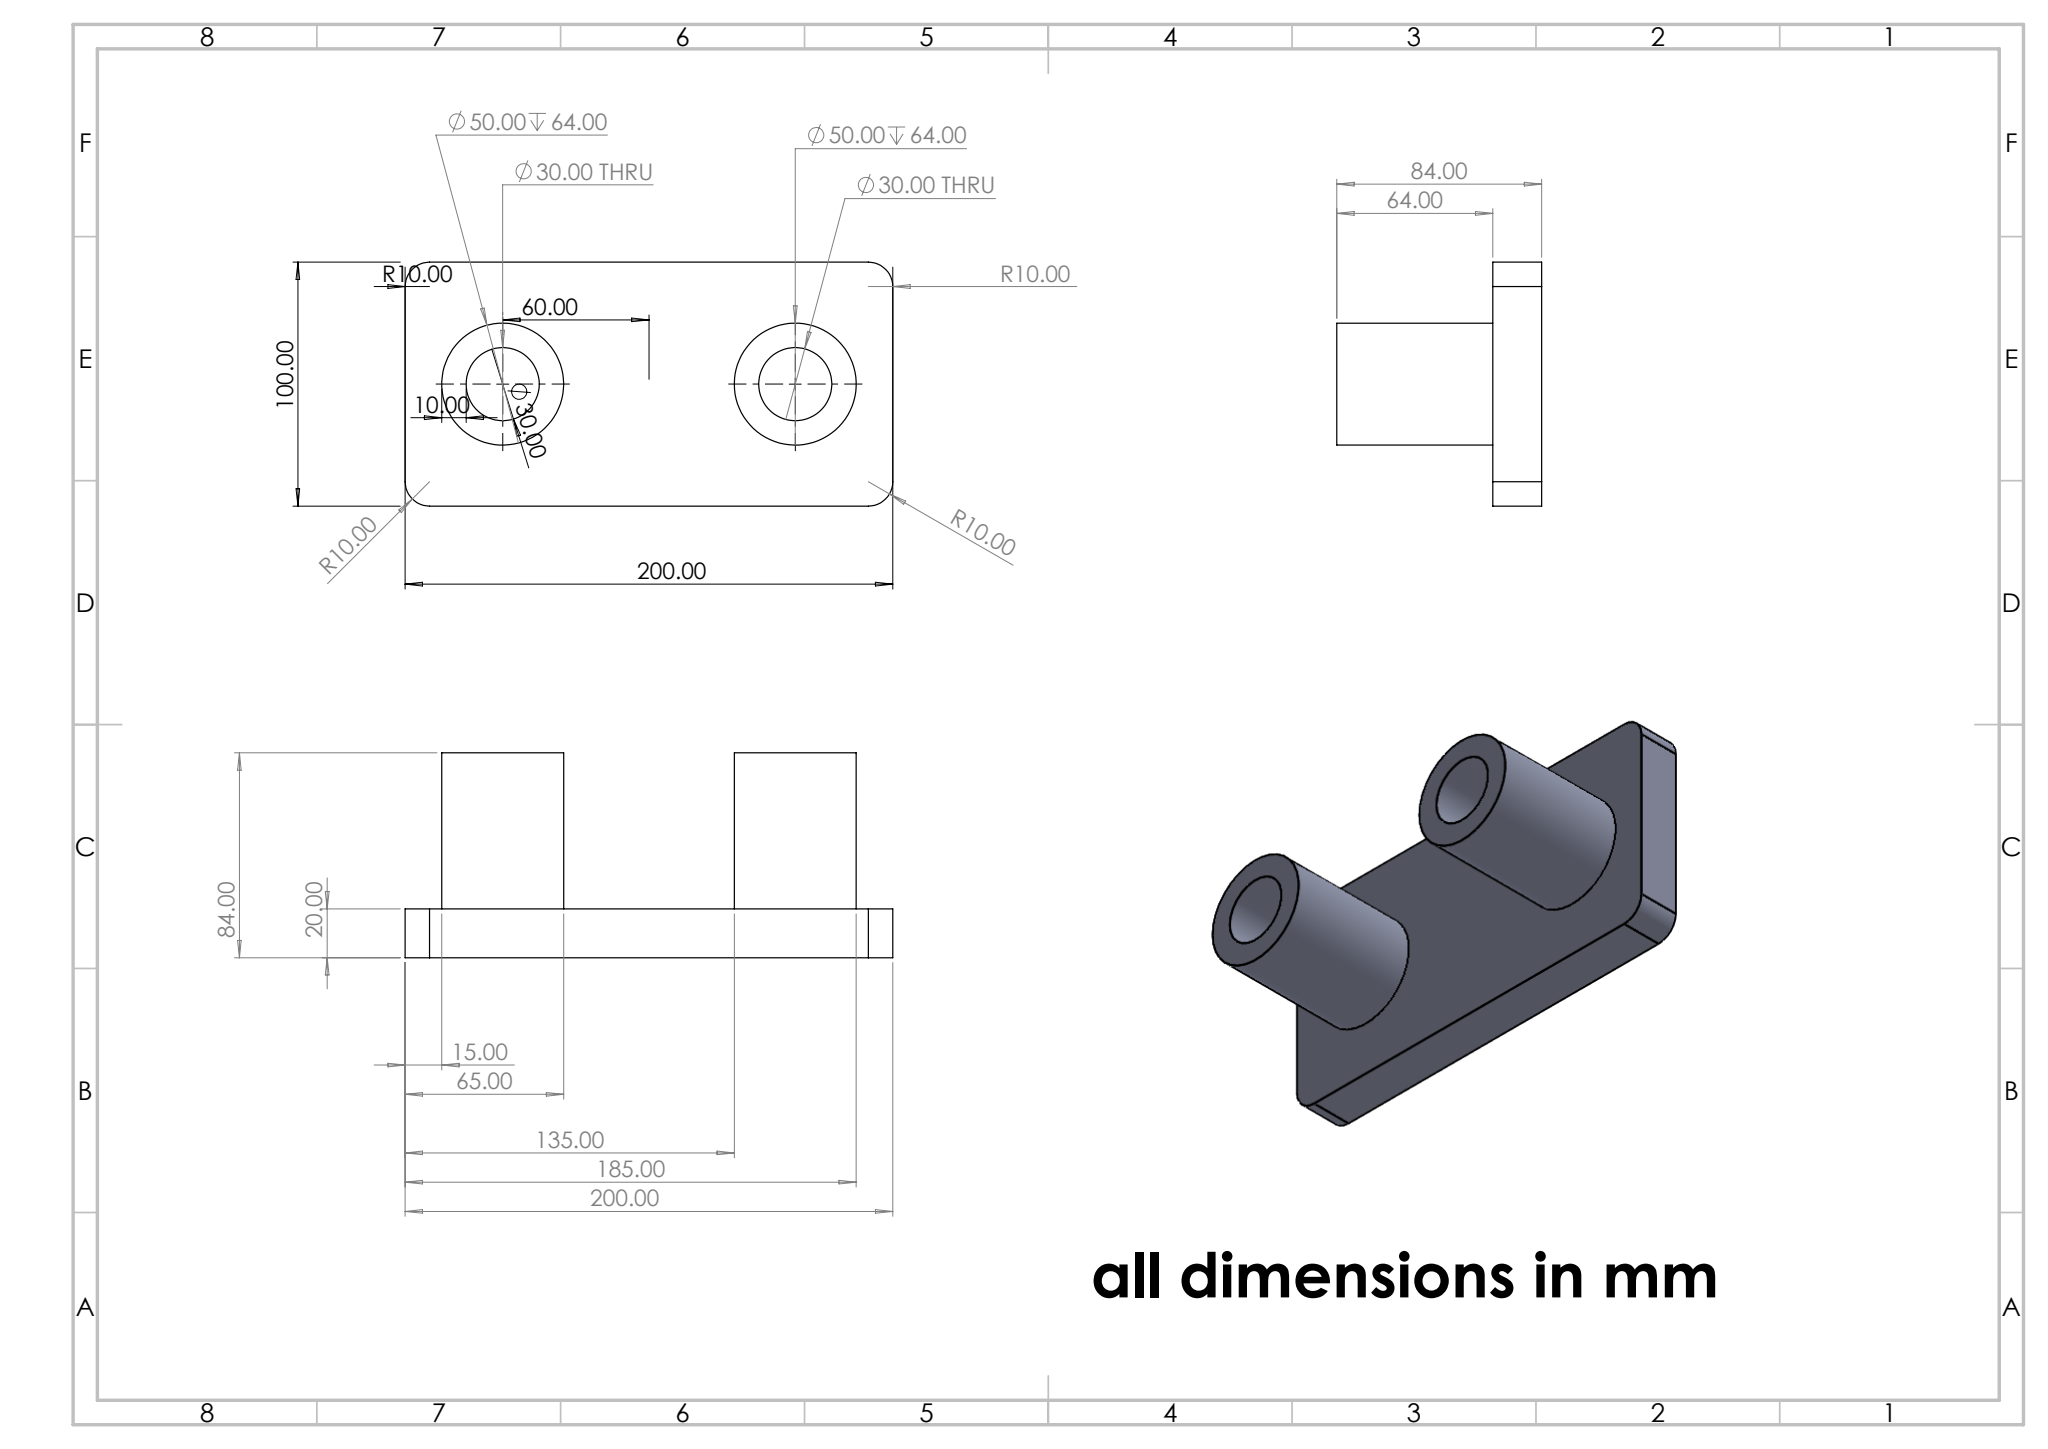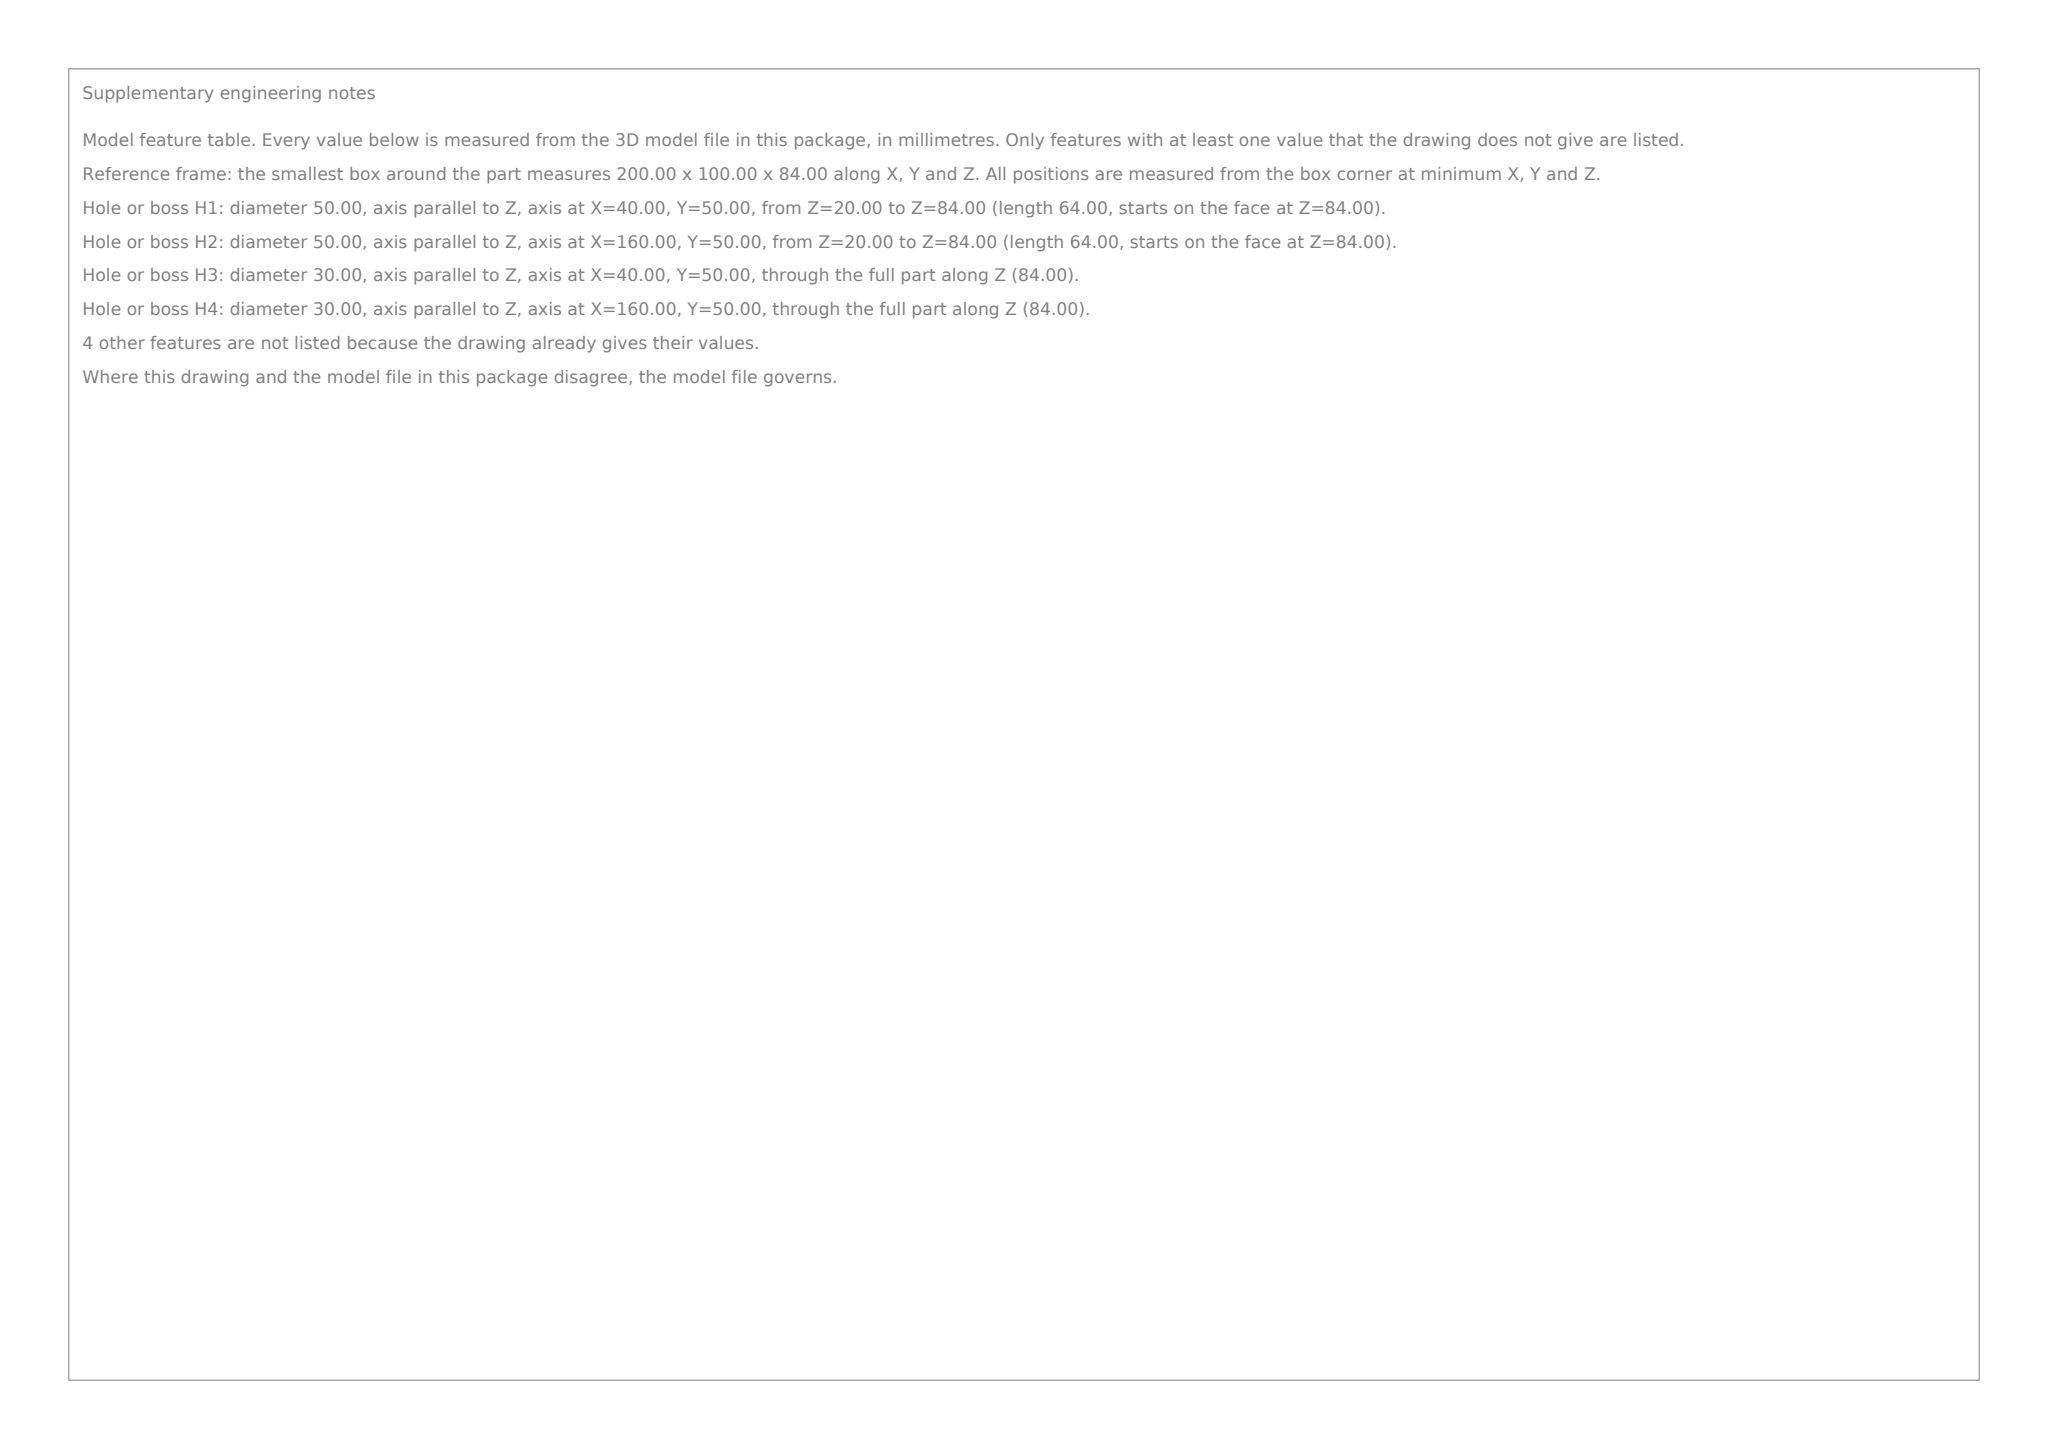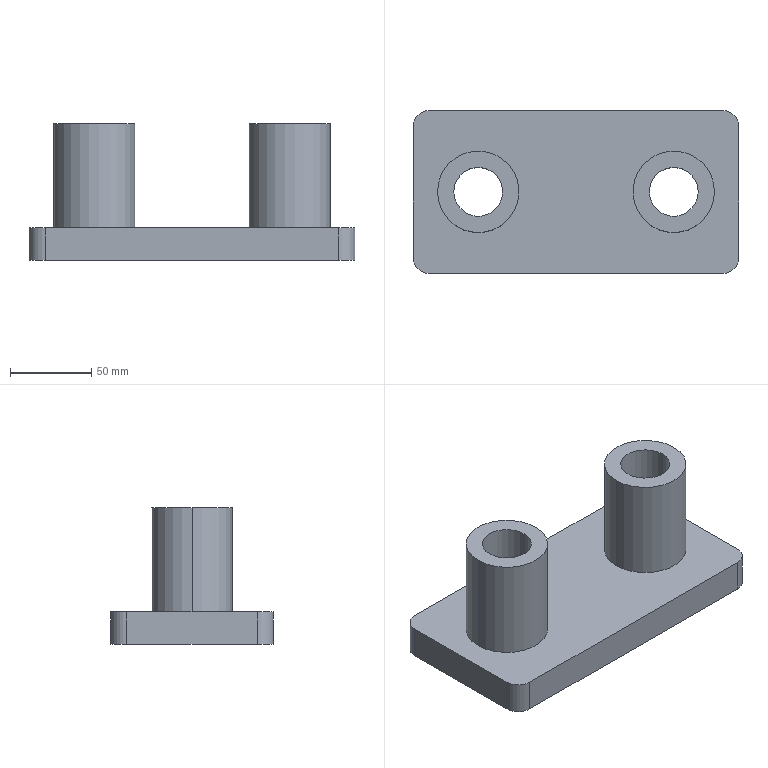Part | SolidWorks | mm | 1 solid | 20 faces | box 200 x 100 x 84 mm | volume 530858 mm3 | cylinder 12 | plane 8 | commonest cylinder face diameters 30 x4 50 x4 20 x4
build123d program:
from build123d import *

# Parameters (mm, degrees)
SKETCH1_W           = 200
SKETCH1_H           = 100
BOSS_EXTRUDE1_DEPTH = 20
SKETCH2_R           = 25
SKETCH2_R_2         = 15
EXTRUDE_THIN1_DEPTH = 64
CUT_EXTRUDE1_START  = -64
SKETCH3_R           = 15
CUT_EXTRUDE1_DEPTH  = 64
FILLET1_R           = 10


with BuildPart() as part:
    # Sketch1 → Boss-Extrude1 (new body)
    with BuildSketch(Plane.XY):
        Rectangle(SKETCH1_W, SKETCH1_H)
    extrude(amount=BOSS_EXTRUDE1_DEPTH)

    # Sketch2 → Extrude-Thin1 (add)
    with BuildSketch(Plane.XY.offset(20)):
        with Locations((-60, 0)):
            Circle(SKETCH2_R)
        with Locations((-60, 0)):
            Circle(SKETCH2_R_2, mode=Mode.SUBTRACT)
    extrude_thin1 = extrude(amount=EXTRUDE_THIN1_DEPTH)

    # Sketch3 → Cut-Extrude1 (cut)
    with BuildSketch(Plane.XY.offset(20).offset(CUT_EXTRUDE1_START)):
        with Locations(Location((-60, 0, 0), (0, 0, 180))):
            Circle(SKETCH3_R)
    cut_extrude1 = extrude(amount=CUT_EXTRUDE1_DEPTH, mode=Mode.SUBTRACT)

    # Mirror1: Extrude-Thin1, Cut-Extrude1 across plane
    add(extrude_thin1.mirror(Plane(origin=(0, 0, 0), x_dir=(0, 0, 1), z_dir=(1, 0, 0))))
    add(cut_extrude1.mirror(Plane(origin=(0, 0, 0), x_dir=(0, 0, 1), z_dir=(1, 0, 0))), mode=Mode.SUBTRACT)

    # Fillet1
    fillet1_edges = [part.edges().sort_by_distance(p)[0] for p in [
        (100, -50, 10),
        (-100, -50, 10),
        (-100, 50, 10),
        (100, 50, 10),
    ]]
    fillet(fillet1_edges, radius=FILLET1_R)


solid = part.part
STEP:
#1=CARTESIAN_POINT('',(75.,0.,84.));
#2=VERTEX_POINT('',#1);
#3=CARTESIAN_POINT('',(45.,0.,84.));
#4=VERTEX_POINT('',#3);
#5=CARTESIAN_POINT('',(60.,0.,84.));
#6=DIRECTION('',(0.,0.,-1.));
#7=DIRECTION('',(-1.,0.,0.));
#8=AXIS2_PLACEMENT_3D('',#5,#6,#7);
#9=CIRCLE('',#8,15.);
#10=EDGE_CURVE('',#2,#4,#9,.T.);
#11=ORIENTED_EDGE('',*,*,#10,.F.);
#12=CARTESIAN_POINT('',(75.,0.,0.));
#13=VERTEX_POINT('',#12);
#14=CARTESIAN_POINT('',(75.,0.,84.));
#15=DIRECTION('',(0.,0.,-1.));
#16=VECTOR('',#15,1000.);
#17=LINE('',#14,#16);
#18=EDGE_CURVE('',#2,#13,#17,.T.);
#19=ORIENTED_EDGE('',*,*,#18,.T.);
#20=CARTESIAN_POINT('',(45.,0.,0.));
#21=VERTEX_POINT('',#20);
#22=CARTESIAN_POINT('',(60.,0.,0.));
#23=DIRECTION('',(0.,0.,1.));
#24=DIRECTION('',(-1.,0.,0.));
#25=AXIS2_PLACEMENT_3D('',#22,#23,#24);
#26=CIRCLE('',#25,15.);
#27=EDGE_CURVE('',#21,#13,#26,.T.);
#28=ORIENTED_EDGE('',*,*,#27,.F.);
#29=CARTESIAN_POINT('',(45.,0.,84.));
#30=DIRECTION('',(0.,0.,-1.));
#31=VECTOR('',#30,1000.);
#32=LINE('',#29,#31);
#33=EDGE_CURVE('',#4,#21,#32,.T.);
#34=ORIENTED_EDGE('',*,*,#33,.F.);
#35=EDGE_LOOP('',(#11,#19,#28,#34));
#36=FACE_OUTER_BOUND('',#35,.T.);
#37=CARTESIAN_POINT('',(60.,0.,84.));
#38=DIRECTION('',(0.,0.,-1.));
#39=DIRECTION('',(-1.,0.,0.));
#40=AXIS2_PLACEMENT_3D('',#37,#38,#39);
#41=CYLINDRICAL_SURFACE('',#40,15.);
#42=ADVANCED_FACE('',(#36),#41,.F.);
#43=CARTESIAN_POINT('',(35.,0.,84.));
#44=VERTEX_POINT('',#43);
#45=CARTESIAN_POINT('',(85.,0.,84.));
#46=VERTEX_POINT('',#45);
#47=CARTESIAN_POINT('',(60.,0.,84.));
#48=DIRECTION('',(0.,0.,-1.));
#49=DIRECTION('',(-1.,0.,0.));
#50=AXIS2_PLACEMENT_3D('',#47,#48,#49);
#51=CIRCLE('',#50,25.);
#52=EDGE_CURVE('',#44,#46,#51,.T.);
#53=ORIENTED_EDGE('',*,*,#52,.T.);
#54=CARTESIAN_POINT('',(85.,0.,20.));
#55=VERTEX_POINT('',#54);
#56=CARTESIAN_POINT('',(85.,0.,84.));
#57=DIRECTION('',(0.,0.,-1.));
#58=VECTOR('',#57,1000.);
#59=LINE('',#56,#58);
#60=EDGE_CURVE('',#46,#55,#59,.T.);
#61=ORIENTED_EDGE('',*,*,#60,.T.);
#62=CARTESIAN_POINT('',(35.,0.,20.));
#63=VERTEX_POINT('',#62);
#64=CARTESIAN_POINT('',(60.,0.,20.));
#65=DIRECTION('',(0.,0.,-1.));
#66=DIRECTION('',(-1.,0.,0.));
#67=AXIS2_PLACEMENT_3D('',#64,#65,#66);
#68=CIRCLE('',#67,25.);
#69=EDGE_CURVE('',#63,#55,#68,.T.);
#70=ORIENTED_EDGE('',*,*,#69,.F.);
#71=CARTESIAN_POINT('',(35.,0.,84.));
#72=DIRECTION('',(0.,0.,-1.));
#73=VECTOR('',#72,1000.);
#74=LINE('',#71,#73);
#75=EDGE_CURVE('',#44,#63,#74,.T.);
#76=ORIENTED_EDGE('',*,*,#75,.F.);
#77=EDGE_LOOP('',(#53,#61,#70,#76));
#78=FACE_OUTER_BOUND('',#77,.T.);
#79=CARTESIAN_POINT('',(60.,0.,84.));
#80=DIRECTION('',(0.,0.,-1.));
#81=DIRECTION('',(-1.,0.,0.));
#82=AXIS2_PLACEMENT_3D('',#79,#80,#81);
#83=CYLINDRICAL_SURFACE('',#82,25.);
#84=ADVANCED_FACE('',(#78),#83,.T.);
#85=CARTESIAN_POINT('',(-75.,0.,84.));
#86=VERTEX_POINT('',#85);
#87=CARTESIAN_POINT('',(-45.,0.,84.));
#88=VERTEX_POINT('',#87);
#89=CARTESIAN_POINT('',(-60.,0.,84.));
#90=DIRECTION('',(0.,0.,1.));
#91=DIRECTION('',(1.,0.,0.));
#92=AXIS2_PLACEMENT_3D('',#89,#90,#91);
#93=CIRCLE('',#92,15.);
#94=EDGE_CURVE('',#86,#88,#93,.T.);
#95=ORIENTED_EDGE('',*,*,#94,.T.);
#96=CARTESIAN_POINT('',(-45.,0.,0.));
#97=VERTEX_POINT('',#96);
#98=CARTESIAN_POINT('',(-45.,0.,84.));
#99=DIRECTION('',(0.,0.,-1.));
#100=VECTOR('',#99,1000.);
#101=LINE('',#98,#100);
#102=EDGE_CURVE('',#88,#97,#101,.T.);
#103=ORIENTED_EDGE('',*,*,#102,.T.);
#104=CARTESIAN_POINT('',(-75.,0.,0.));
#105=VERTEX_POINT('',#104);
#106=CARTESIAN_POINT('',(-60.,0.,0.));
#107=DIRECTION('',(0.,0.,-1.));
#108=DIRECTION('',(-1.,0.,0.));
#109=AXIS2_PLACEMENT_3D('',#106,#107,#108);
#110=CIRCLE('',#109,15.);
#111=EDGE_CURVE('',#97,#105,#110,.T.);
#112=ORIENTED_EDGE('',*,*,#111,.T.);
#113=CARTESIAN_POINT('',(-75.,0.,84.));
#114=DIRECTION('',(0.,0.,-1.));
#115=VECTOR('',#114,1000.);
#116=LINE('',#113,#115);
#117=EDGE_CURVE('',#86,#105,#116,.T.);
#118=ORIENTED_EDGE('',*,*,#117,.F.);
#119=EDGE_LOOP('',(#95,#103,#112,#118));
#120=FACE_OUTER_BOUND('',#119,.T.);
#121=CARTESIAN_POINT('',(-60.,0.,84.));
#122=DIRECTION('',(0.,0.,-1.));
#123=DIRECTION('',(-1.,0.,0.));
#124=AXIS2_PLACEMENT_3D('',#121,#122,#123);
#125=CYLINDRICAL_SURFACE('',#124,15.);
#126=ADVANCED_FACE('',(#120),#125,.F.);
#127=CARTESIAN_POINT('',(-35.,0.,84.));
#128=VERTEX_POINT('',#127);
#129=CARTESIAN_POINT('',(-85.,0.,84.));
#130=VERTEX_POINT('',#129);
#131=CARTESIAN_POINT('',(-60.,0.,84.));
#132=DIRECTION('',(0.,0.,1.));
#133=DIRECTION('',(1.,0.,0.));
#134=AXIS2_PLACEMENT_3D('',#131,#132,#133);
#135=CIRCLE('',#134,25.);
#136=EDGE_CURVE('',#128,#130,#135,.T.);
#137=ORIENTED_EDGE('',*,*,#136,.F.);
#138=CARTESIAN_POINT('',(-35.,0.,20.));
#139=VERTEX_POINT('',#138);
#140=CARTESIAN_POINT('',(-35.,0.,84.));
#141=DIRECTION('',(0.,0.,-1.));
#142=VECTOR('',#141,1000.);
#143=LINE('',#140,#142);
#144=EDGE_CURVE('',#128,#139,#143,.T.);
#145=ORIENTED_EDGE('',*,*,#144,.T.);
#146=CARTESIAN_POINT('',(-85.,0.,20.));
#147=VERTEX_POINT('',#146);
#148=CARTESIAN_POINT('',(-60.,0.,20.));
#149=DIRECTION('',(0.,0.,1.));
#150=DIRECTION('',(-1.,0.,0.));
#151=AXIS2_PLACEMENT_3D('',#148,#149,#150);
#152=CIRCLE('',#151,25.);
#153=EDGE_CURVE('',#139,#147,#152,.T.);
#154=ORIENTED_EDGE('',*,*,#153,.T.);
#155=CARTESIAN_POINT('',(-85.,0.,84.));
#156=DIRECTION('',(0.,0.,-1.));
#157=VECTOR('',#156,1000.);
#158=LINE('',#155,#157);
#159=EDGE_CURVE('',#130,#147,#158,.T.);
#160=ORIENTED_EDGE('',*,*,#159,.F.);
#161=EDGE_LOOP('',(#137,#145,#154,#160));
#162=FACE_OUTER_BOUND('',#161,.T.);
#163=CARTESIAN_POINT('',(-60.,0.,84.));
#164=DIRECTION('',(0.,0.,-1.));
#165=DIRECTION('',(-1.,0.,0.));
#166=AXIS2_PLACEMENT_3D('',#163,#164,#165);
#167=CYLINDRICAL_SURFACE('',#166,25.);
#168=ADVANCED_FACE('',(#162),#167,.T.);
#169=CARTESIAN_POINT('',(100.,-40.,20.));
#170=VERTEX_POINT('',#169);
#171=CARTESIAN_POINT('',(100.,40.,20.));
#172=VERTEX_POINT('',#171);
#173=CARTESIAN_POINT('',(100.,-50.,20.));
#174=DIRECTION('',(0.,1.,0.));
#175=VECTOR('',#174,1000.);
#176=LINE('',#173,#175);
#177=EDGE_CURVE('',#170,#172,#176,.T.);
#178=ORIENTED_EDGE('',*,*,#177,.F.);
#179=CARTESIAN_POINT('',(100.,-40.,0.));
#180=VERTEX_POINT('',#179);
#181=CARTESIAN_POINT('',(100.,-40.,20.));
#182=DIRECTION('',(0.,0.,-1.));
#183=VECTOR('',#182,1000.);
#184=LINE('',#181,#183);
#185=EDGE_CURVE('',#170,#180,#184,.T.);
#186=ORIENTED_EDGE('',*,*,#185,.T.);
#187=CARTESIAN_POINT('',(100.,40.,0.));
#188=VERTEX_POINT('',#187);
#189=CARTESIAN_POINT('',(100.,-50.,0.));
#190=DIRECTION('',(0.,1.,0.));
#191=VECTOR('',#190,1000.);
#192=LINE('',#189,#191);
#193=EDGE_CURVE('',#180,#188,#192,.T.);
#194=ORIENTED_EDGE('',*,*,#193,.T.);
#195=CARTESIAN_POINT('',(100.,40.,20.));
#196=DIRECTION('',(0.,0.,1.));
#197=VECTOR('',#196,1000.);
#198=LINE('',#195,#197);
#199=EDGE_CURVE('',#188,#172,#198,.T.);
#200=ORIENTED_EDGE('',*,*,#199,.T.);
#201=EDGE_LOOP('',(#178,#186,#194,#200));
#202=FACE_OUTER_BOUND('',#201,.T.);
#203=CARTESIAN_POINT('',(100.,-50.,20.));
#204=DIRECTION('',(-1.,0.,0.));
#205=DIRECTION('',(0.,0.,1.));
#206=AXIS2_PLACEMENT_3D('',#203,#204,#205);
#207=PLANE('',#206);
#208=ADVANCED_FACE('',(#202),#207,.F.);
#209=CARTESIAN_POINT('',(90.,50.,20.));
#210=VERTEX_POINT('',#209);
#211=CARTESIAN_POINT('',(-90.,50.,20.));
#212=VERTEX_POINT('',#211);
#213=CARTESIAN_POINT('',(-100.,50.,20.));
#214=DIRECTION('',(-1.,0.,0.));
#215=VECTOR('',#214,1000.);
#216=LINE('',#213,#215);
#217=EDGE_CURVE('',#210,#212,#216,.T.);
#218=ORIENTED_EDGE('',*,*,#217,.F.);
#219=CARTESIAN_POINT('',(90.,50.,0.));
#220=VERTEX_POINT('',#219);
#221=CARTESIAN_POINT('',(90.,50.,20.));
#222=DIRECTION('',(0.,0.,-1.));
#223=VECTOR('',#222,1000.);
#224=LINE('',#221,#223);
#225=EDGE_CURVE('',#210,#220,#224,.T.);
#226=ORIENTED_EDGE('',*,*,#225,.T.);
#227=CARTESIAN_POINT('',(-90.,50.,0.));
#228=VERTEX_POINT('',#227);
#229=CARTESIAN_POINT('',(-100.,50.,0.));
#230=DIRECTION('',(-1.,0.,0.));
#231=VECTOR('',#230,1000.);
#232=LINE('',#229,#231);
#233=EDGE_CURVE('',#220,#228,#232,.T.);
#234=ORIENTED_EDGE('',*,*,#233,.T.);
#235=CARTESIAN_POINT('',(-90.,50.,20.));
#236=DIRECTION('',(0.,0.,1.));
#237=VECTOR('',#236,1000.);
#238=LINE('',#235,#237);
#239=EDGE_CURVE('',#228,#212,#238,.T.);
#240=ORIENTED_EDGE('',*,*,#239,.T.);
#241=EDGE_LOOP('',(#218,#226,#234,#240));
#242=FACE_OUTER_BOUND('',#241,.T.);
#243=CARTESIAN_POINT('',(-100.,50.,20.));
#244=DIRECTION('',(0.,-1.,0.));
#245=DIRECTION('',(0.,0.,-1.));
#246=AXIS2_PLACEMENT_3D('',#243,#244,#245);
#247=PLANE('',#246);
#248=ADVANCED_FACE('',(#242),#247,.F.);
#249=CARTESIAN_POINT('',(-100.,40.,0.));
#250=VERTEX_POINT('',#249);
#251=CARTESIAN_POINT('',(-100.,-40.,0.));
#252=VERTEX_POINT('',#251);
#253=CARTESIAN_POINT('',(-100.,-50.,0.));
#254=DIRECTION('',(0.,-1.,0.));
#255=VECTOR('',#254,1000.);
#256=LINE('',#253,#255);
#257=EDGE_CURVE('',#250,#252,#256,.T.);
#258=ORIENTED_EDGE('',*,*,#257,.T.);
#259=CARTESIAN_POINT('',(-100.,-40.,20.));
#260=VERTEX_POINT('',#259);
#261=CARTESIAN_POINT('',(-100.,-40.,20.));
#262=DIRECTION('',(0.,0.,1.));
#263=VECTOR('',#262,1000.);
#264=LINE('',#261,#263);
#265=EDGE_CURVE('',#252,#260,#264,.T.);
#266=ORIENTED_EDGE('',*,*,#265,.T.);
#267=CARTESIAN_POINT('',(-100.,40.,20.));
#268=VERTEX_POINT('',#267);
#269=CARTESIAN_POINT('',(-100.,-50.,20.));
#270=DIRECTION('',(0.,-1.,0.));
#271=VECTOR('',#270,1000.);
#272=LINE('',#269,#271);
#273=EDGE_CURVE('',#268,#260,#272,.T.);
#274=ORIENTED_EDGE('',*,*,#273,.F.);
#275=CARTESIAN_POINT('',(-100.,40.,20.));
#276=DIRECTION('',(0.,0.,-1.));
#277=VECTOR('',#276,1000.);
#278=LINE('',#275,#277);
#279=EDGE_CURVE('',#268,#250,#278,.T.);
#280=ORIENTED_EDGE('',*,*,#279,.T.);
#281=EDGE_LOOP('',(#258,#266,#274,#280));
#282=FACE_OUTER_BOUND('',#281,.T.);
#283=CARTESIAN_POINT('',(-100.,-50.,20.));
#284=DIRECTION('',(1.,0.,0.));
#285=DIRECTION('',(0.,0.,-1.));
#286=AXIS2_PLACEMENT_3D('',#283,#284,#285);
#287=PLANE('',#286);
#288=ADVANCED_FACE('',(#282),#287,.F.);
#289=CARTESIAN_POINT('',(-90.,-50.,0.));
#290=VERTEX_POINT('',#289);
#291=CARTESIAN_POINT('',(90.,-50.,0.));
#292=VERTEX_POINT('',#291);
#293=CARTESIAN_POINT('',(-100.,-50.,0.));
#294=DIRECTION('',(1.,0.,0.));
#295=VECTOR('',#294,1000.);
#296=LINE('',#293,#295);
#297=EDGE_CURVE('',#290,#292,#296,.T.);
#298=ORIENTED_EDGE('',*,*,#297,.T.);
#299=CARTESIAN_POINT('',(90.,-50.,20.));
#300=VERTEX_POINT('',#299);
#301=CARTESIAN_POINT('',(90.,-50.,20.));
#302=DIRECTION('',(0.,0.,1.));
#303=VECTOR('',#302,1000.);
#304=LINE('',#301,#303);
#305=EDGE_CURVE('',#292,#300,#304,.T.);
#306=ORIENTED_EDGE('',*,*,#305,.T.);
#307=CARTESIAN_POINT('',(-90.,-50.,20.));
#308=VERTEX_POINT('',#307);
#309=CARTESIAN_POINT('',(-100.,-50.,20.));
#310=DIRECTION('',(1.,0.,0.));
#311=VECTOR('',#310,1000.);
#312=LINE('',#309,#311);
#313=EDGE_CURVE('',#308,#300,#312,.T.);
#314=ORIENTED_EDGE('',*,*,#313,.F.);
#315=CARTESIAN_POINT('',(-90.,-50.,20.));
#316=DIRECTION('',(0.,0.,-1.));
#317=VECTOR('',#316,1000.);
#318=LINE('',#315,#317);
#319=EDGE_CURVE('',#308,#290,#318,.T.);
#320=ORIENTED_EDGE('',*,*,#319,.T.);
#321=EDGE_LOOP('',(#298,#306,#314,#320));
#322=FACE_OUTER_BOUND('',#321,.T.);
#323=CARTESIAN_POINT('',(-100.,-50.,20.));
#324=DIRECTION('',(0.,1.,0.));
#325=DIRECTION('',(0.,0.,1.));
#326=AXIS2_PLACEMENT_3D('',#323,#324,#325);
#327=PLANE('',#326);
#328=ADVANCED_FACE('',(#322),#327,.F.);
#329=ORIENTED_EDGE('',*,*,#69,.T.);
#330=CARTESIAN_POINT('',(60.,0.,20.));
#331=DIRECTION('',(0.,0.,-1.));
#332=DIRECTION('',(-1.,0.,0.));
#333=AXIS2_PLACEMENT_3D('',#330,#331,#332);
#334=CIRCLE('',#333,25.);
#335=EDGE_CURVE('',#55,#63,#334,.T.);
#336=ORIENTED_EDGE('',*,*,#335,.T.);
#337=EDGE_LOOP('',(#329,#336));
#338=FACE_BOUND('',#337,.T.);
#339=CARTESIAN_POINT('',(-60.,0.,20.));
#340=DIRECTION('',(0.,0.,1.));
#341=DIRECTION('',(-1.,0.,0.));
#342=AXIS2_PLACEMENT_3D('',#339,#340,#341);
#343=CIRCLE('',#342,25.);
#344=EDGE_CURVE('',#147,#139,#343,.T.);
#345=ORIENTED_EDGE('',*,*,#344,.F.);
#346=ORIENTED_EDGE('',*,*,#153,.F.);
#347=EDGE_LOOP('',(#345,#346));
#348=FACE_BOUND('',#347,.T.);
#349=ORIENTED_EDGE('',*,*,#313,.T.);
#350=CARTESIAN_POINT('',(90.,-40.,20.));
#351=DIRECTION('',(0.,0.,1.));
#352=DIRECTION('',(-1.,0.,0.));
#353=AXIS2_PLACEMENT_3D('',#350,#351,#352);
#354=CIRCLE('',#353,10.);
#355=EDGE_CURVE('',#300,#170,#354,.T.);
#356=ORIENTED_EDGE('',*,*,#355,.T.);
#357=ORIENTED_EDGE('',*,*,#177,.T.);
#358=CARTESIAN_POINT('',(90.,40.,20.));
#359=DIRECTION('',(0.,0.,1.));
#360=DIRECTION('',(-1.,0.,0.));
#361=AXIS2_PLACEMENT_3D('',#358,#359,#360);
#362=CIRCLE('',#361,10.);
#363=EDGE_CURVE('',#172,#210,#362,.T.);
#364=ORIENTED_EDGE('',*,*,#363,.T.);
#365=ORIENTED_EDGE('',*,*,#217,.T.);
#366=CARTESIAN_POINT('',(-90.,40.,20.));
#367=DIRECTION('',(0.,0.,1.));
#368=DIRECTION('',(-1.,0.,0.));
#369=AXIS2_PLACEMENT_3D('',#366,#367,#368);
#370=CIRCLE('',#369,10.);
#371=EDGE_CURVE('',#212,#268,#370,.T.);
#372=ORIENTED_EDGE('',*,*,#371,.T.);
#373=ORIENTED_EDGE('',*,*,#273,.T.);
#374=CARTESIAN_POINT('',(-90.,-40.,20.));
#375=DIRECTION('',(0.,0.,1.));
#376=DIRECTION('',(-1.,0.,0.));
#377=AXIS2_PLACEMENT_3D('',#374,#375,#376);
#378=CIRCLE('',#377,10.);
#379=EDGE_CURVE('',#260,#308,#378,.T.);
#380=ORIENTED_EDGE('',*,*,#379,.T.);
#381=EDGE_LOOP('',(#349,#356,#357,#364,#365,#372,#373,#380));
#382=FACE_OUTER_BOUND('',#381,.T.);
#383=CARTESIAN_POINT('',(0.,0.,20.));
#384=DIRECTION('',(0.,0.,-1.));
#385=DIRECTION('',(-1.,0.,0.));
#386=AXIS2_PLACEMENT_3D('',#383,#384,#385);
#387=PLANE('',#386);
#388=ADVANCED_FACE('',(#338,#348,#382),#387,.F.);
#389=ORIENTED_EDGE('',*,*,#27,.T.);
#390=CARTESIAN_POINT('',(60.,0.,0.));
#391=DIRECTION('',(0.,0.,1.));
#392=DIRECTION('',(-1.,0.,0.));
#393=AXIS2_PLACEMENT_3D('',#390,#391,#392);
#394=CIRCLE('',#393,15.);
#395=EDGE_CURVE('',#13,#21,#394,.T.);
#396=ORIENTED_EDGE('',*,*,#395,.T.);
#397=EDGE_LOOP('',(#389,#396));
#398=FACE_BOUND('',#397,.T.);
#399=CARTESIAN_POINT('',(-60.,0.,0.));
#400=DIRECTION('',(0.,0.,-1.));
#401=DIRECTION('',(-1.,0.,0.));
#402=AXIS2_PLACEMENT_3D('',#399,#400,#401);
#403=CIRCLE('',#402,15.);
#404=EDGE_CURVE('',#105,#97,#403,.T.);
#405=ORIENTED_EDGE('',*,*,#404,.F.);
#406=ORIENTED_EDGE('',*,*,#111,.F.);
#407=EDGE_LOOP('',(#405,#406));
#408=FACE_BOUND('',#407,.T.);
#409=ORIENTED_EDGE('',*,*,#193,.F.);
#410=CARTESIAN_POINT('',(90.,-40.,0.));
#411=DIRECTION('',(0.,0.,-1.));
#412=DIRECTION('',(-1.,0.,0.));
#413=AXIS2_PLACEMENT_3D('',#410,#411,#412);
#414=CIRCLE('',#413,10.);
#415=EDGE_CURVE('',#180,#292,#414,.T.);
#416=ORIENTED_EDGE('',*,*,#415,.T.);
#417=ORIENTED_EDGE('',*,*,#297,.F.);
#418=CARTESIAN_POINT('',(-90.,-40.,0.));
#419=DIRECTION('',(0.,0.,-1.));
#420=DIRECTION('',(-1.,0.,0.));
#421=AXIS2_PLACEMENT_3D('',#418,#419,#420);
#422=CIRCLE('',#421,10.);
#423=EDGE_CURVE('',#290,#252,#422,.T.);
#424=ORIENTED_EDGE('',*,*,#423,.T.);
#425=ORIENTED_EDGE('',*,*,#257,.F.);
#426=CARTESIAN_POINT('',(-90.,40.,0.));
#427=DIRECTION('',(0.,0.,-1.));
#428=DIRECTION('',(-1.,0.,0.));
#429=AXIS2_PLACEMENT_3D('',#426,#427,#428);
#430=CIRCLE('',#429,10.);
#431=EDGE_CURVE('',#250,#228,#430,.T.);
#432=ORIENTED_EDGE('',*,*,#431,.T.);
#433=ORIENTED_EDGE('',*,*,#233,.F.);
#434=CARTESIAN_POINT('',(90.,40.,0.));
#435=DIRECTION('',(0.,0.,-1.));
#436=DIRECTION('',(-1.,0.,0.));
#437=AXIS2_PLACEMENT_3D('',#434,#435,#436);
#438=CIRCLE('',#437,10.);
#439=EDGE_CURVE('',#220,#188,#438,.T.);
#440=ORIENTED_EDGE('',*,*,#439,.T.);
#441=EDGE_LOOP('',(#409,#416,#417,#424,#425,#432,#433,#440));
#442=FACE_OUTER_BOUND('',#441,.T.);
#443=CARTESIAN_POINT('',(0.,0.,0.));
#444=DIRECTION('',(0.,0.,-1.));
#445=DIRECTION('',(-1.,0.,0.));
#446=AXIS2_PLACEMENT_3D('',#443,#444,#445);
#447=PLANE('',#446);
#448=ADVANCED_FACE('',(#398,#408,#442),#447,.T.);
#449=CARTESIAN_POINT('',(-60.,0.,84.));
#450=DIRECTION('',(0.,0.,1.));
#451=DIRECTION('',(1.,0.,0.));
#452=AXIS2_PLACEMENT_3D('',#449,#450,#451);
#453=CIRCLE('',#452,25.);
#454=EDGE_CURVE('',#130,#128,#453,.T.);
#455=ORIENTED_EDGE('',*,*,#454,.T.);
#456=ORIENTED_EDGE('',*,*,#136,.T.);
#457=EDGE_LOOP('',(#455,#456));
#458=FACE_OUTER_BOUND('',#457,.T.);
#459=ORIENTED_EDGE('',*,*,#94,.F.);
#460=CARTESIAN_POINT('',(-60.,0.,84.));
#461=DIRECTION('',(0.,0.,1.));
#462=DIRECTION('',(1.,0.,0.));
#463=AXIS2_PLACEMENT_3D('',#460,#461,#462);
#464=CIRCLE('',#463,15.);
#465=EDGE_CURVE('',#88,#86,#464,.T.);
#466=ORIENTED_EDGE('',*,*,#465,.F.);
#467=EDGE_LOOP('',(#459,#466));
#468=FACE_BOUND('',#467,.T.);
#469=CARTESIAN_POINT('',(-60.,0.,84.));
#470=DIRECTION('',(0.,0.,1.));
#471=DIRECTION('',(1.,0.,0.));
#472=AXIS2_PLACEMENT_3D('',#469,#470,#471);
#473=PLANE('',#472);
#474=ADVANCED_FACE('',(#458,#468),#473,.T.);
#475=ORIENTED_EDGE('',*,*,#144,.F.);
#476=ORIENTED_EDGE('',*,*,#454,.F.);
#477=ORIENTED_EDGE('',*,*,#159,.T.);
#478=ORIENTED_EDGE('',*,*,#344,.T.);
#479=EDGE_LOOP('',(#475,#476,#477,#478));
#480=FACE_OUTER_BOUND('',#479,.T.);
#481=CARTESIAN_POINT('',(-60.,0.,84.));
#482=DIRECTION('',(0.,0.,-1.));
#483=DIRECTION('',(-1.,0.,0.));
#484=AXIS2_PLACEMENT_3D('',#481,#482,#483);
#485=CYLINDRICAL_SURFACE('',#484,25.);
#486=ADVANCED_FACE('',(#480),#485,.T.);
#487=ORIENTED_EDGE('',*,*,#102,.F.);
#488=ORIENTED_EDGE('',*,*,#465,.T.);
#489=ORIENTED_EDGE('',*,*,#117,.T.);
#490=ORIENTED_EDGE('',*,*,#404,.T.);
#491=EDGE_LOOP('',(#487,#488,#489,#490));
#492=FACE_OUTER_BOUND('',#491,.T.);
#493=CARTESIAN_POINT('',(-60.,0.,84.));
#494=DIRECTION('',(0.,0.,-1.));
#495=DIRECTION('',(-1.,0.,0.));
#496=AXIS2_PLACEMENT_3D('',#493,#494,#495);
#497=CYLINDRICAL_SURFACE('',#496,15.);
#498=ADVANCED_FACE('',(#492),#497,.F.);
#499=ORIENTED_EDGE('',*,*,#60,.F.);
#500=CARTESIAN_POINT('',(60.,0.,84.));
#501=DIRECTION('',(0.,0.,-1.));
#502=DIRECTION('',(-1.,0.,0.));
#503=AXIS2_PLACEMENT_3D('',#500,#501,#502);
#504=CIRCLE('',#503,25.);
#505=EDGE_CURVE('',#46,#44,#504,.T.);
#506=ORIENTED_EDGE('',*,*,#505,.T.);
#507=ORIENTED_EDGE('',*,*,#75,.T.);
#508=ORIENTED_EDGE('',*,*,#335,.F.);
#509=EDGE_LOOP('',(#499,#506,#507,#508));
#510=FACE_OUTER_BOUND('',#509,.T.);
#511=CARTESIAN_POINT('',(60.,0.,84.));
#512=DIRECTION('',(0.,0.,-1.));
#513=DIRECTION('',(-1.,0.,0.));
#514=AXIS2_PLACEMENT_3D('',#511,#512,#513);
#515=CYLINDRICAL_SURFACE('',#514,25.);
#516=ADVANCED_FACE('',(#510),#515,.T.);
#517=CARTESIAN_POINT('',(60.,0.,84.));
#518=DIRECTION('',(0.,0.,-1.));
#519=DIRECTION('',(-1.,0.,0.));
#520=AXIS2_PLACEMENT_3D('',#517,#518,#519);
#521=CIRCLE('',#520,15.);
#522=EDGE_CURVE('',#4,#2,#521,.T.);
#523=ORIENTED_EDGE('',*,*,#522,.T.);
#524=ORIENTED_EDGE('',*,*,#10,.T.);
#525=EDGE_LOOP('',(#523,#524));
#526=FACE_BOUND('',#525,.T.);
#527=ORIENTED_EDGE('',*,*,#52,.F.);
#528=ORIENTED_EDGE('',*,*,#505,.F.);
#529=EDGE_LOOP('',(#527,#528));
#530=FACE_OUTER_BOUND('',#529,.T.);
#531=CARTESIAN_POINT('',(60.,0.,84.));
#532=DIRECTION('',(0.,0.,-1.));
#533=DIRECTION('',(-1.,0.,0.));
#534=AXIS2_PLACEMENT_3D('',#531,#532,#533);
#535=PLANE('',#534);
#536=ADVANCED_FACE('',(#526,#530),#535,.F.);
#537=ORIENTED_EDGE('',*,*,#18,.F.);
#538=ORIENTED_EDGE('',*,*,#522,.F.);
#539=ORIENTED_EDGE('',*,*,#33,.T.);
#540=ORIENTED_EDGE('',*,*,#395,.F.);
#541=EDGE_LOOP('',(#537,#538,#539,#540));
#542=FACE_OUTER_BOUND('',#541,.T.);
#543=CARTESIAN_POINT('',(60.,0.,84.));
#544=DIRECTION('',(0.,0.,-1.));
#545=DIRECTION('',(-1.,0.,0.));
#546=AXIS2_PLACEMENT_3D('',#543,#544,#545);
#547=CYLINDRICAL_SURFACE('',#546,15.);
#548=ADVANCED_FACE('',(#542),#547,.F.);
#549=ORIENTED_EDGE('',*,*,#355,.F.);
#550=ORIENTED_EDGE('',*,*,#305,.F.);
#551=ORIENTED_EDGE('',*,*,#415,.F.);
#552=ORIENTED_EDGE('',*,*,#185,.F.);
#553=EDGE_LOOP('',(#549,#550,#551,#552));
#554=FACE_OUTER_BOUND('',#553,.T.);
#555=CARTESIAN_POINT('',(90.,-40.,20.));
#556=DIRECTION('',(0.,0.,-1.));
#557=DIRECTION('',(-1.,0.,0.));
#558=AXIS2_PLACEMENT_3D('',#555,#556,#557);
#559=CYLINDRICAL_SURFACE('',#558,10.);
#560=ADVANCED_FACE('',(#554),#559,.T.);
#561=ORIENTED_EDGE('',*,*,#379,.F.);
#562=ORIENTED_EDGE('',*,*,#265,.F.);
#563=ORIENTED_EDGE('',*,*,#423,.F.);
#564=ORIENTED_EDGE('',*,*,#319,.F.);
#565=EDGE_LOOP('',(#561,#562,#563,#564));
#566=FACE_OUTER_BOUND('',#565,.T.);
#567=CARTESIAN_POINT('',(-90.,-40.,20.));
#568=DIRECTION('',(0.,0.,-1.));
#569=DIRECTION('',(-1.,0.,0.));
#570=AXIS2_PLACEMENT_3D('',#567,#568,#569);
#571=CYLINDRICAL_SURFACE('',#570,10.);
#572=ADVANCED_FACE('',(#566),#571,.T.);
#573=ORIENTED_EDGE('',*,*,#363,.F.);
#574=ORIENTED_EDGE('',*,*,#199,.F.);
#575=ORIENTED_EDGE('',*,*,#439,.F.);
#576=ORIENTED_EDGE('',*,*,#225,.F.);
#577=EDGE_LOOP('',(#573,#574,#575,#576));
#578=FACE_OUTER_BOUND('',#577,.T.);
#579=CARTESIAN_POINT('',(90.,40.,20.));
#580=DIRECTION('',(0.,0.,-1.));
#581=DIRECTION('',(-1.,0.,0.));
#582=AXIS2_PLACEMENT_3D('',#579,#580,#581);
#583=CYLINDRICAL_SURFACE('',#582,10.);
#584=ADVANCED_FACE('',(#578),#583,.T.);
#585=ORIENTED_EDGE('',*,*,#371,.F.);
#586=ORIENTED_EDGE('',*,*,#239,.F.);
#587=ORIENTED_EDGE('',*,*,#431,.F.);
#588=ORIENTED_EDGE('',*,*,#279,.F.);
#589=EDGE_LOOP('',(#585,#586,#587,#588));
#590=FACE_OUTER_BOUND('',#589,.T.);
#591=CARTESIAN_POINT('',(-90.,40.,20.));
#592=DIRECTION('',(0.,0.,-1.));
#593=DIRECTION('',(-1.,0.,0.));
#594=AXIS2_PLACEMENT_3D('',#591,#592,#593);
#595=CYLINDRICAL_SURFACE('',#594,10.);
#596=ADVANCED_FACE('',(#590),#595,.T.);
#597=CLOSED_SHELL('',(#42,#84,#126,#168,#208,#248,#288,#328,#388,#448,#474,#486,#498,#516,#536,#548,#560,#572,#584,#596));
#598=MANIFOLD_SOLID_BREP('',#597);
#599=CARTESIAN_POINT('',(0.,0.,0.));
#600=DIRECTION('',(0.,0.,1.));
#601=DIRECTION('',(1.,0.,0.));
#602=AXIS2_PLACEMENT_3D('',#599,#600,#601);
#603=(LENGTH_UNIT()NAMED_UNIT(*)SI_UNIT(.MILLI.,.METRE.));
#604=UNCERTAINTY_MEASURE_WITH_UNIT(LENGTH_MEASURE(0.00001),#603,'','');
#605=(NAMED_UNIT(*)PLANE_ANGLE_UNIT()SI_UNIT($,.RADIAN.));
#606=(NAMED_UNIT(*)SI_UNIT($,.STERADIAN.)SOLID_ANGLE_UNIT());
#607=(GEOMETRIC_REPRESENTATION_CONTEXT(3)GLOBAL_UNCERTAINTY_ASSIGNED_CONTEXT((#604))GLOBAL_UNIT_ASSIGNED_CONTEXT((#603,#605,#606))REPRESENTATION_CONTEXT('',''));
#608=ADVANCED_BREP_SHAPE_REPRESENTATION('',(#598,#602),#607);